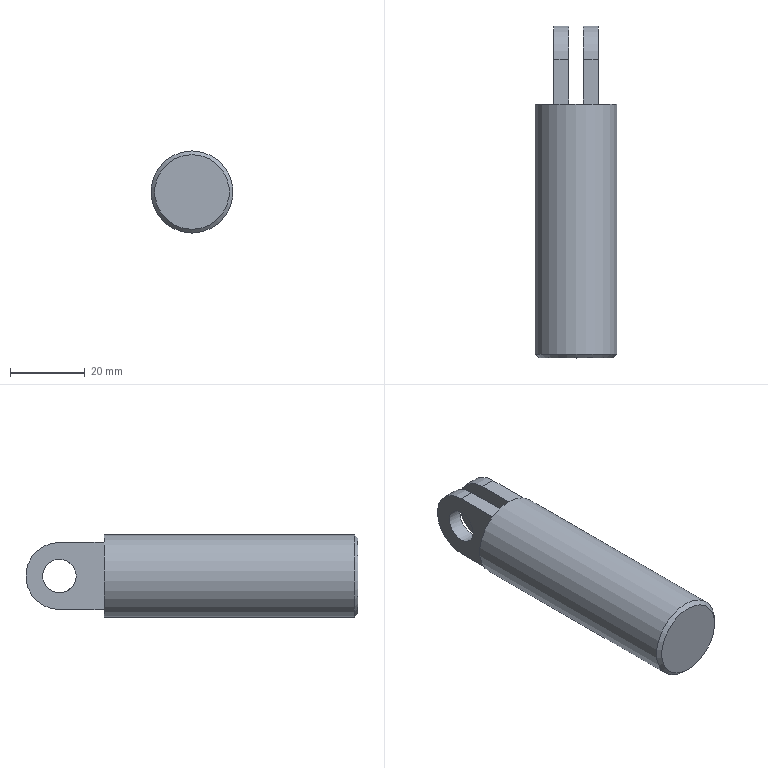Component | NX | PLUNGER | 1 solid | 16 faces | box 22 x 89 x 22 mm | volume 28052 mm3 | plane 10 | cylinder 5 | cone 1 | commonest cylinder face diameters 18 x2 9 x2 22 x1
STEP:
#1=CARTESIAN_POINT('',(0.,0.,0.));
#2=DIRECTION('',(0.,0.,1.));
#3=DIRECTION('',(1.,0.,0.));
#4=AXIS2_PLACEMENT_3D('',#1,#2,#3);
#5=CARTESIAN_POINT('',(-2.,64.5,19.75));
#6=VERTEX_POINT('',#5);
#7=CARTESIAN_POINT('',(-2.,52.5,19.75));
#8=VERTEX_POINT('',#7);
#9=CARTESIAN_POINT('',(-2.,64.5,19.75));
#10=DIRECTION('',(0.,-1.,-0.));
#11=VECTOR('',#10,1.);
#12=LINE('',#9,#11);
#13=CARTESIAN_POINT('',(-6.,64.5,19.75));
#14=DIRECTION('',(0.,-0.,1.));
#15=DIRECTION('',(0.,-1.,-0.));
#16=AXIS2_PLACEMENT_3D('',#13,#14,#15);
#17=PLANE('',#16);
#18=CARTESIAN_POINT('',(0.,4.));
#19=DIRECTION('',(1.,0.));
#20=VECTOR('',#19,1.);
#21=LINE('',#18,#20);
#22=(GEOMETRIC_REPRESENTATION_CONTEXT(2)PARAMETRIC_REPRESENTATION_CONTEXT()REPRESENTATION_CONTEXT('',''));
#23=DEFINITIONAL_REPRESENTATION('',(#21),#22);
#24=PCURVE('',#17,#23);
#25=CARTESIAN_POINT('',(-2.,76.,27.55));
#26=DIRECTION('',(-1.,0.,0.));
#27=DIRECTION('',(0.,-1.,0.));
#28=AXIS2_PLACEMENT_3D('',#25,#26,#27);
#29=PLANE('',#28);
#30=CARTESIAN_POINT('',(11.5,-7.8));
#31=DIRECTION('',(1.,-0.));
#32=VECTOR('',#31,1.);
#33=LINE('',#30,#32);
#34=(GEOMETRIC_REPRESENTATION_CONTEXT(2)PARAMETRIC_REPRESENTATION_CONTEXT()REPRESENTATION_CONTEXT('',''));
#35=DEFINITIONAL_REPRESENTATION('',(#33),#34);
#36=PCURVE('',#29,#35);
#37=SURFACE_CURVE('',#12,(#24,#36),.PCURVE_S1.);
#38=EDGE_CURVE('',#6,#8,#37,.T.);
#39=ORIENTED_EDGE('',*,*,#38,.F.);
#40=CARTESIAN_POINT('',(-6.,64.5,19.75));
#41=VERTEX_POINT('',#40);
#42=CARTESIAN_POINT('',(-6.,64.5,19.75));
#43=DIRECTION('',(1.,0.,0.));
#44=VECTOR('',#43,1.);
#45=LINE('',#42,#44);
#46=CARTESIAN_POINT('',(0.,0.));
#47=DIRECTION('',(0.,1.));
#48=VECTOR('',#47,1.);
#49=LINE('',#46,#48);
#50=(GEOMETRIC_REPRESENTATION_CONTEXT(2)PARAMETRIC_REPRESENTATION_CONTEXT()REPRESENTATION_CONTEXT('',''));
#51=DEFINITIONAL_REPRESENTATION('',(#49),#50);
#52=PCURVE('',#17,#51);
#53=CARTESIAN_POINT('',(-6.,64.5,10.75));
#54=DIRECTION('',(1.,0.,0.));
#55=DIRECTION('',(0.,1.,0.));
#56=AXIS2_PLACEMENT_3D('',#53,#54,#55);
#57=CYLINDRICAL_SURFACE('',#56,9.);
#58=CARTESIAN_POINT('',(7.854,0.));
#59=DIRECTION('',(0.,1.));
#60=VECTOR('',#59,1.);
#61=LINE('',#58,#60);
#62=(GEOMETRIC_REPRESENTATION_CONTEXT(2)PARAMETRIC_REPRESENTATION_CONTEXT()REPRESENTATION_CONTEXT('',''));
#63=DEFINITIONAL_REPRESENTATION('',(#61),#62);
#64=PCURVE('',#57,#63);
#65=SURFACE_CURVE('',#45,(#52,#64),.PCURVE_S1.);
#66=EDGE_CURVE('',#41,#6,#65,.T.);
#67=ORIENTED_EDGE('',*,*,#66,.F.);
#68=CARTESIAN_POINT('',(-6.,52.5,19.75));
#69=VERTEX_POINT('',#68);
#70=CARTESIAN_POINT('',(-6.,64.5,19.75));
#71=DIRECTION('',(0.,-1.,-0.));
#72=VECTOR('',#71,1.);
#73=LINE('',#70,#72);
#74=CARTESIAN_POINT('',(0.,0.));
#75=DIRECTION('',(1.,0.));
#76=VECTOR('',#75,1.);
#77=LINE('',#74,#76);
#78=(GEOMETRIC_REPRESENTATION_CONTEXT(2)PARAMETRIC_REPRESENTATION_CONTEXT()REPRESENTATION_CONTEXT('',''));
#79=DEFINITIONAL_REPRESENTATION('',(#77),#78);
#80=PCURVE('',#17,#79);
#81=CARTESIAN_POINT('',(-6.,64.5,10.75));
#82=DIRECTION('',(1.,0.,0.));
#83=DIRECTION('',(0.,1.,0.));
#84=AXIS2_PLACEMENT_3D('',#81,#82,#83);
#85=PLANE('',#84);
#86=CARTESIAN_POINT('',(0.,9.));
#87=DIRECTION('',(-1.,-0.));
#88=VECTOR('',#87,1.);
#89=LINE('',#86,#88);
#90=(GEOMETRIC_REPRESENTATION_CONTEXT(2)PARAMETRIC_REPRESENTATION_CONTEXT()REPRESENTATION_CONTEXT('',''));
#91=DEFINITIONAL_REPRESENTATION('',(#89),#90);
#92=PCURVE('',#85,#91);
#93=SURFACE_CURVE('',#73,(#80,#92),.PCURVE_S1.);
#94=EDGE_CURVE('',#41,#69,#93,.T.);
#95=ORIENTED_EDGE('',*,*,#94,.T.);
#96=CARTESIAN_POINT('',(-6.,52.5,19.75));
#97=DIRECTION('',(1.,0.,0.));
#98=VECTOR('',#97,1.);
#99=LINE('',#96,#98);
#100=CARTESIAN_POINT('',(12.,0.));
#101=DIRECTION('',(0.,1.));
#102=VECTOR('',#101,1.);
#103=LINE('',#100,#102);
#104=(GEOMETRIC_REPRESENTATION_CONTEXT(2)PARAMETRIC_REPRESENTATION_CONTEXT()REPRESENTATION_CONTEXT('',''));
#105=DEFINITIONAL_REPRESENTATION('',(#103),#104);
#106=PCURVE('',#17,#105);
#107=CARTESIAN_POINT('',(-0.,52.5,10.75));
#108=DIRECTION('',(0.,1.,0.));
#109=DIRECTION('',(0.,0.,1.));
#110=AXIS2_PLACEMENT_3D('',#107,#108,#109);
#111=PLANE('',#110);
#112=CARTESIAN_POINT('',(9.,-6.));
#113=DIRECTION('',(0.,1.));
#114=VECTOR('',#113,1.);
#115=LINE('',#112,#114);
#116=(GEOMETRIC_REPRESENTATION_CONTEXT(2)PARAMETRIC_REPRESENTATION_CONTEXT()REPRESENTATION_CONTEXT('',''));
#117=DEFINITIONAL_REPRESENTATION('',(#115),#116);
#118=PCURVE('',#111,#117);
#119=SURFACE_CURVE('',#99,(#106,#118),.PCURVE_S1.);
#120=EDGE_CURVE('',#69,#8,#119,.T.);
#121=ORIENTED_EDGE('',*,*,#120,.T.);
#122=EDGE_LOOP('',(#39,#67,#95,#121));
#123=FACE_BOUND('',#122,.T.);
#124=ADVANCED_FACE('',(#123),#17,.T.);
#125=CARTESIAN_POINT('',(-2.,52.5,1.75));
#126=VERTEX_POINT('',#125);
#127=CARTESIAN_POINT('',(-2.,64.5,1.75));
#128=VERTEX_POINT('',#127);
#129=CARTESIAN_POINT('',(-2.,52.5,1.75));
#130=DIRECTION('',(0.,1.,-0.));
#131=VECTOR('',#130,1.);
#132=LINE('',#129,#131);
#133=CARTESIAN_POINT('',(-6.,52.5,1.75));
#134=DIRECTION('',(0.,-0.,-1.));
#135=DIRECTION('',(0.,1.,-0.));
#136=AXIS2_PLACEMENT_3D('',#133,#134,#135);
#137=PLANE('',#136);
#138=CARTESIAN_POINT('',(0.,4.));
#139=DIRECTION('',(1.,0.));
#140=VECTOR('',#139,1.);
#141=LINE('',#138,#140);
#142=(GEOMETRIC_REPRESENTATION_CONTEXT(2)PARAMETRIC_REPRESENTATION_CONTEXT()REPRESENTATION_CONTEXT('',''));
#143=DEFINITIONAL_REPRESENTATION('',(#141),#142);
#144=PCURVE('',#137,#143);
#145=CARTESIAN_POINT('',(23.5,-25.8));
#146=DIRECTION('',(-1.,-0.));
#147=VECTOR('',#146,1.);
#148=LINE('',#145,#147);
#149=(GEOMETRIC_REPRESENTATION_CONTEXT(2)PARAMETRIC_REPRESENTATION_CONTEXT()REPRESENTATION_CONTEXT('',''));
#150=DEFINITIONAL_REPRESENTATION('',(#148),#149);
#151=PCURVE('',#29,#150);
#152=SURFACE_CURVE('',#132,(#144,#151),.PCURVE_S1.);
#153=EDGE_CURVE('',#126,#128,#152,.T.);
#154=ORIENTED_EDGE('',*,*,#153,.F.);
#155=CARTESIAN_POINT('',(-6.,52.5,1.75));
#156=VERTEX_POINT('',#155);
#157=CARTESIAN_POINT('',(-6.,52.5,1.75));
#158=DIRECTION('',(1.,0.,0.));
#159=VECTOR('',#158,1.);
#160=LINE('',#157,#159);
#161=CARTESIAN_POINT('',(0.,0.));
#162=DIRECTION('',(0.,1.));
#163=VECTOR('',#162,1.);
#164=LINE('',#161,#163);
#165=(GEOMETRIC_REPRESENTATION_CONTEXT(2)PARAMETRIC_REPRESENTATION_CONTEXT()REPRESENTATION_CONTEXT('',''));
#166=DEFINITIONAL_REPRESENTATION('',(#164),#165);
#167=PCURVE('',#137,#166);
#168=CARTESIAN_POINT('',(-9.,-6.));
#169=DIRECTION('',(0.,1.));
#170=VECTOR('',#169,1.);
#171=LINE('',#168,#170);
#172=(GEOMETRIC_REPRESENTATION_CONTEXT(2)PARAMETRIC_REPRESENTATION_CONTEXT()REPRESENTATION_CONTEXT('',''));
#173=DEFINITIONAL_REPRESENTATION('',(#171),#172);
#174=PCURVE('',#111,#173);
#175=SURFACE_CURVE('',#160,(#167,#174),.PCURVE_S1.);
#176=EDGE_CURVE('',#156,#126,#175,.T.);
#177=ORIENTED_EDGE('',*,*,#176,.F.);
#178=CARTESIAN_POINT('',(-6.,64.5,1.75));
#179=VERTEX_POINT('',#178);
#180=CARTESIAN_POINT('',(-6.,52.5,1.75));
#181=DIRECTION('',(0.,1.,-0.));
#182=VECTOR('',#181,1.);
#183=LINE('',#180,#182);
#184=CARTESIAN_POINT('',(0.,0.));
#185=DIRECTION('',(1.,0.));
#186=VECTOR('',#185,1.);
#187=LINE('',#184,#186);
#188=(GEOMETRIC_REPRESENTATION_CONTEXT(2)PARAMETRIC_REPRESENTATION_CONTEXT()REPRESENTATION_CONTEXT('',''));
#189=DEFINITIONAL_REPRESENTATION('',(#187),#188);
#190=PCURVE('',#137,#189);
#191=CARTESIAN_POINT('',(-12.,-9.));
#192=DIRECTION('',(1.,-0.));
#193=VECTOR('',#192,1.);
#194=LINE('',#191,#193);
#195=(GEOMETRIC_REPRESENTATION_CONTEXT(2)PARAMETRIC_REPRESENTATION_CONTEXT()REPRESENTATION_CONTEXT('',''));
#196=DEFINITIONAL_REPRESENTATION('',(#194),#195);
#197=PCURVE('',#85,#196);
#198=SURFACE_CURVE('',#183,(#190,#197),.PCURVE_S1.);
#199=EDGE_CURVE('',#156,#179,#198,.T.);
#200=ORIENTED_EDGE('',*,*,#199,.T.);
#201=CARTESIAN_POINT('',(-6.,64.5,1.75));
#202=DIRECTION('',(1.,0.,0.));
#203=VECTOR('',#202,1.);
#204=LINE('',#201,#203);
#205=CARTESIAN_POINT('',(12.,0.));
#206=DIRECTION('',(0.,1.));
#207=VECTOR('',#206,1.);
#208=LINE('',#205,#207);
#209=(GEOMETRIC_REPRESENTATION_CONTEXT(2)PARAMETRIC_REPRESENTATION_CONTEXT()REPRESENTATION_CONTEXT('',''));
#210=DEFINITIONAL_REPRESENTATION('',(#208),#209);
#211=PCURVE('',#137,#210);
#212=CARTESIAN_POINT('',(4.712,0.));
#213=DIRECTION('',(0.,1.));
#214=VECTOR('',#213,1.);
#215=LINE('',#212,#214);
#216=(GEOMETRIC_REPRESENTATION_CONTEXT(2)PARAMETRIC_REPRESENTATION_CONTEXT()REPRESENTATION_CONTEXT('',''));
#217=DEFINITIONAL_REPRESENTATION('',(#215),#216);
#218=PCURVE('',#57,#217);
#219=SURFACE_CURVE('',#204,(#211,#218),.PCURVE_S1.);
#220=EDGE_CURVE('',#179,#128,#219,.T.);
#221=ORIENTED_EDGE('',*,*,#220,.T.);
#222=EDGE_LOOP('',(#154,#177,#200,#221));
#223=FACE_BOUND('',#222,.T.);
#224=ADVANCED_FACE('',(#223),#137,.T.);
#225=CARTESIAN_POINT('',(-2.,64.5,10.75));
#226=DIRECTION('',(1.,0.,0.));
#227=DIRECTION('',(0.,-1.,0.));
#228=AXIS2_PLACEMENT_3D('',#225,#226,#227);
#229=CIRCLE('',#228,9.);
#230=CARTESIAN_POINT('',(3.142,4.));
#231=DIRECTION('',(1.,0.));
#232=VECTOR('',#231,1.);
#233=LINE('',#230,#232);
#234=(GEOMETRIC_REPRESENTATION_CONTEXT(2)PARAMETRIC_REPRESENTATION_CONTEXT()REPRESENTATION_CONTEXT('',''));
#235=DEFINITIONAL_REPRESENTATION('',(#233),#234);
#236=PCURVE('',#57,#235);
#237=CARTESIAN_POINT('',(20.5,-16.8));
#238=CARTESIAN_POINT('',(20.5,-32.388));
#239=CARTESIAN_POINT('',(7.,-24.594));
#240=CARTESIAN_POINT('',(-6.5,-16.8));
#241=CARTESIAN_POINT('',(7.,-9.006));
#242=CARTESIAN_POINT('',(20.5,-1.212));
#243=CARTESIAN_POINT('',(20.5,-16.8));
#244=(BOUNDED_CURVE()B_SPLINE_CURVE(2,(#237,#238,#239,#240,#241,#242,#243),.UNSPECIFIED.,.T.,.F.)B_SPLINE_CURVE_WITH_KNOTS((1,2,2,2,2,1),(-2.094,0.,2.094,4.189,6.283,8.378),.UNSPECIFIED.)CURVE()GEOMETRIC_REPRESENTATION_ITEM()RATIONAL_B_SPLINE_CURVE((1.,0.5,1.,0.5,1.,0.5,1.))REPRESENTATION_ITEM(''));
#245=(GEOMETRIC_REPRESENTATION_CONTEXT(2)PARAMETRIC_REPRESENTATION_CONTEXT()REPRESENTATION_CONTEXT('',''));
#246=DEFINITIONAL_REPRESENTATION('',(#244),#245);
#247=PCURVE('',#29,#246);
#248=SURFACE_CURVE('',#229,(#236,#247),.PCURVE_S1.);
#249=EDGE_CURVE('',#128,#6,#248,.T.);
#250=ORIENTED_EDGE('',*,*,#249,.F.);
#251=ORIENTED_EDGE('',*,*,#220,.F.);
#252=CARTESIAN_POINT('',(-6.,64.5,10.75));
#253=DIRECTION('',(1.,0.,0.));
#254=DIRECTION('',(0.,0.,1.));
#255=AXIS2_PLACEMENT_3D('',#252,#253,#254);
#256=CIRCLE('',#255,9.);
#257=CARTESIAN_POINT('',(1.571,0.));
#258=DIRECTION('',(1.,0.));
#259=VECTOR('',#258,1.);
#260=LINE('',#257,#259);
#261=(GEOMETRIC_REPRESENTATION_CONTEXT(2)PARAMETRIC_REPRESENTATION_CONTEXT()REPRESENTATION_CONTEXT('',''));
#262=DEFINITIONAL_REPRESENTATION('',(#260),#261);
#263=PCURVE('',#57,#262);
#264=CARTESIAN_POINT('',(0.,0.));
#265=DIRECTION('',(0.,1.));
#266=AXIS2_PLACEMENT_2D('',#264,#265);
#267=CIRCLE('',#266,9.);
#268=(GEOMETRIC_REPRESENTATION_CONTEXT(2)PARAMETRIC_REPRESENTATION_CONTEXT()REPRESENTATION_CONTEXT('',''));
#269=DEFINITIONAL_REPRESENTATION('',(#267),#268);
#270=PCURVE('',#85,#269);
#271=SURFACE_CURVE('',#256,(#263,#270),.PCURVE_S1.);
#272=EDGE_CURVE('',#179,#41,#271,.T.);
#273=ORIENTED_EDGE('',*,*,#272,.T.);
#274=ORIENTED_EDGE('',*,*,#66,.T.);
#275=EDGE_LOOP('',(#250,#251,#273,#274));
#276=FACE_BOUND('',#275,.T.);
#277=ADVANCED_FACE('',(#276),#57,.T.);
#278=CARTESIAN_POINT('',(2.,52.5,19.75));
#279=VERTEX_POINT('',#278);
#280=CARTESIAN_POINT('',(6.,52.5,19.75));
#281=VERTEX_POINT('',#280);
#282=CARTESIAN_POINT('',(-6.,52.5,19.75));
#283=DIRECTION('',(1.,0.,0.));
#284=VECTOR('',#283,1.);
#285=LINE('',#282,#284);
#286=CARTESIAN_POINT('',(9.,-6.));
#287=DIRECTION('',(0.,1.));
#288=VECTOR('',#287,1.);
#289=LINE('',#286,#288);
#290=(GEOMETRIC_REPRESENTATION_CONTEXT(2)PARAMETRIC_REPRESENTATION_CONTEXT()REPRESENTATION_CONTEXT('',''));
#291=DEFINITIONAL_REPRESENTATION('',(#289),#290);
#292=PCURVE('',#111,#291);
#293=CARTESIAN_POINT('',(-6.,64.5,19.75));
#294=DIRECTION('',(0.,-0.,1.));
#295=DIRECTION('',(0.,-1.,-0.));
#296=AXIS2_PLACEMENT_3D('',#293,#294,#295);
#297=PLANE('',#296);
#298=CARTESIAN_POINT('',(12.,0.));
#299=DIRECTION('',(0.,1.));
#300=VECTOR('',#299,1.);
#301=LINE('',#298,#300);
#302=(GEOMETRIC_REPRESENTATION_CONTEXT(2)PARAMETRIC_REPRESENTATION_CONTEXT()REPRESENTATION_CONTEXT('',''));
#303=DEFINITIONAL_REPRESENTATION('',(#301),#302);
#304=PCURVE('',#297,#303);
#305=SURFACE_CURVE('',#285,(#292,#304),.PCURVE_S1.);
#306=EDGE_CURVE('',#279,#281,#305,.T.);
#307=ORIENTED_EDGE('',*,*,#306,.F.);
#308=CARTESIAN_POINT('',(2.,52.5,1.75));
#309=VERTEX_POINT('',#308);
#310=CARTESIAN_POINT('',(2.,52.5,-6.05));
#311=DIRECTION('',(0.,0.,1.));
#312=VECTOR('',#311,1.);
#313=LINE('',#310,#312);
#314=CARTESIAN_POINT('',(-16.8,2.));
#315=DIRECTION('',(1.,0.));
#316=VECTOR('',#315,1.);
#317=LINE('',#314,#316);
#318=(GEOMETRIC_REPRESENTATION_CONTEXT(2)PARAMETRIC_REPRESENTATION_CONTEXT()REPRESENTATION_CONTEXT('',''));
#319=DEFINITIONAL_REPRESENTATION('',(#317),#318);
#320=PCURVE('',#111,#319);
#321=CARTESIAN_POINT('',(2.,76.,-6.05));
#322=DIRECTION('',(1.,0.,0.));
#323=DIRECTION('',(0.,1.,0.));
#324=AXIS2_PLACEMENT_3D('',#321,#322,#323);
#325=PLANE('',#324);
#326=CARTESIAN_POINT('',(-23.5,0.));
#327=DIRECTION('',(0.,1.));
#328=VECTOR('',#327,1.);
#329=LINE('',#326,#328);
#330=(GEOMETRIC_REPRESENTATION_CONTEXT(2)PARAMETRIC_REPRESENTATION_CONTEXT()REPRESENTATION_CONTEXT('',''));
#331=DEFINITIONAL_REPRESENTATION('',(#329),#330);
#332=PCURVE('',#325,#331);
#333=SURFACE_CURVE('',#313,(#320,#332),.PCURVE_S1.);
#334=EDGE_CURVE('',#309,#279,#333,.T.);
#335=ORIENTED_EDGE('',*,*,#334,.F.);
#336=CARTESIAN_POINT('',(6.,52.5,1.75));
#337=VERTEX_POINT('',#336);
#338=CARTESIAN_POINT('',(-6.,52.5,1.75));
#339=DIRECTION('',(1.,0.,0.));
#340=VECTOR('',#339,1.);
#341=LINE('',#338,#340);
#342=CARTESIAN_POINT('',(-9.,-6.));
#343=DIRECTION('',(0.,1.));
#344=VECTOR('',#343,1.);
#345=LINE('',#342,#344);
#346=(GEOMETRIC_REPRESENTATION_CONTEXT(2)PARAMETRIC_REPRESENTATION_CONTEXT()REPRESENTATION_CONTEXT('',''));
#347=DEFINITIONAL_REPRESENTATION('',(#345),#346);
#348=PCURVE('',#111,#347);
#349=CARTESIAN_POINT('',(-6.,52.5,1.75));
#350=DIRECTION('',(0.,-0.,-1.));
#351=DIRECTION('',(0.,1.,-0.));
#352=AXIS2_PLACEMENT_3D('',#349,#350,#351);
#353=PLANE('',#352);
#354=CARTESIAN_POINT('',(0.,0.));
#355=DIRECTION('',(0.,1.));
#356=VECTOR('',#355,1.);
#357=LINE('',#354,#356);
#358=(GEOMETRIC_REPRESENTATION_CONTEXT(2)PARAMETRIC_REPRESENTATION_CONTEXT()REPRESENTATION_CONTEXT('',''));
#359=DEFINITIONAL_REPRESENTATION('',(#357),#358);
#360=PCURVE('',#353,#359);
#361=SURFACE_CURVE('',#341,(#348,#360),.PCURVE_S1.);
#362=EDGE_CURVE('',#309,#337,#361,.T.);
#363=ORIENTED_EDGE('',*,*,#362,.T.);
#364=CARTESIAN_POINT('',(6.,52.5,10.75));
#365=DIRECTION('',(0.,0.,-1.));
#366=VECTOR('',#365,1.);
#367=LINE('',#364,#366);
#368=CARTESIAN_POINT('',(0.,6.));
#369=DIRECTION('',(-1.,0.));
#370=VECTOR('',#369,1.);
#371=LINE('',#368,#370);
#372=(GEOMETRIC_REPRESENTATION_CONTEXT(2)PARAMETRIC_REPRESENTATION_CONTEXT()REPRESENTATION_CONTEXT('',''));
#373=DEFINITIONAL_REPRESENTATION('',(#371),#372);
#374=PCURVE('',#111,#373);
#375=CARTESIAN_POINT('',(6.,64.5,10.75));
#376=DIRECTION('',(1.,0.,0.));
#377=DIRECTION('',(0.,1.,0.));
#378=AXIS2_PLACEMENT_3D('',#375,#376,#377);
#379=PLANE('',#378);
#380=CARTESIAN_POINT('',(-12.,0.));
#381=DIRECTION('',(0.,-1.));
#382=VECTOR('',#381,1.);
#383=LINE('',#380,#382);
#384=(GEOMETRIC_REPRESENTATION_CONTEXT(2)PARAMETRIC_REPRESENTATION_CONTEXT()REPRESENTATION_CONTEXT('',''));
#385=DEFINITIONAL_REPRESENTATION('',(#383),#384);
#386=PCURVE('',#379,#385);
#387=SURFACE_CURVE('',#367,(#374,#386),.PCURVE_S1.);
#388=EDGE_CURVE('',#281,#337,#387,.T.);
#389=ORIENTED_EDGE('',*,*,#388,.F.);
#390=EDGE_LOOP('',(#307,#335,#363,#389));
#391=FACE_BOUND('',#390,.T.);
#392=CARTESIAN_POINT('',(-2.,52.5,27.55));
#393=DIRECTION('',(0.,0.,-1.));
#394=VECTOR('',#393,1.);
#395=LINE('',#392,#394);
#396=CARTESIAN_POINT('',(16.8,-2.));
#397=DIRECTION('',(-1.,0.));
#398=VECTOR('',#397,1.);
#399=LINE('',#396,#398);
#400=(GEOMETRIC_REPRESENTATION_CONTEXT(2)PARAMETRIC_REPRESENTATION_CONTEXT()REPRESENTATION_CONTEXT('',''));
#401=DEFINITIONAL_REPRESENTATION('',(#399),#400);
#402=PCURVE('',#111,#401);
#403=CARTESIAN_POINT('',(23.5,0.));
#404=DIRECTION('',(0.,-1.));
#405=VECTOR('',#404,1.);
#406=LINE('',#403,#405);
#407=(GEOMETRIC_REPRESENTATION_CONTEXT(2)PARAMETRIC_REPRESENTATION_CONTEXT()REPRESENTATION_CONTEXT('',''));
#408=DEFINITIONAL_REPRESENTATION('',(#406),#407);
#409=PCURVE('',#29,#408);
#410=SURFACE_CURVE('',#395,(#402,#409),.PCURVE_S1.);
#411=EDGE_CURVE('',#8,#126,#410,.T.);
#412=ORIENTED_EDGE('',*,*,#411,.F.);
#413=ORIENTED_EDGE('',*,*,#120,.F.);
#414=CARTESIAN_POINT('',(-6.,52.5,19.75));
#415=DIRECTION('',(0.,0.,-1.));
#416=VECTOR('',#415,1.);
#417=LINE('',#414,#416);
#418=CARTESIAN_POINT('',(9.,-6.));
#419=DIRECTION('',(-1.,0.));
#420=VECTOR('',#419,1.);
#421=LINE('',#418,#420);
#422=(GEOMETRIC_REPRESENTATION_CONTEXT(2)PARAMETRIC_REPRESENTATION_CONTEXT()REPRESENTATION_CONTEXT('',''));
#423=DEFINITIONAL_REPRESENTATION('',(#421),#422);
#424=PCURVE('',#111,#423);
#425=CARTESIAN_POINT('',(-12.,9.));
#426=DIRECTION('',(0.,-1.));
#427=VECTOR('',#426,1.);
#428=LINE('',#425,#427);
#429=(GEOMETRIC_REPRESENTATION_CONTEXT(2)PARAMETRIC_REPRESENTATION_CONTEXT()REPRESENTATION_CONTEXT('',''));
#430=DEFINITIONAL_REPRESENTATION('',(#428),#429);
#431=PCURVE('',#85,#430);
#432=SURFACE_CURVE('',#417,(#424,#431),.PCURVE_S1.);
#433=EDGE_CURVE('',#69,#156,#432,.T.);
#434=ORIENTED_EDGE('',*,*,#433,.T.);
#435=ORIENTED_EDGE('',*,*,#176,.T.);
#436=EDGE_LOOP('',(#412,#413,#434,#435));
#437=FACE_BOUND('',#436,.T.);
#438=CARTESIAN_POINT('',(-0.,52.5,21.75));
#439=VERTEX_POINT('',#438);
#440=CARTESIAN_POINT('',(-0.,52.5,10.75));
#441=DIRECTION('',(0.,-1.,0.));
#442=DIRECTION('',(0.,0.,1.));
#443=AXIS2_PLACEMENT_3D('',#440,#441,#442);
#444=CIRCLE('',#443,11.);
#445=CARTESIAN_POINT('',(11.,0.));
#446=CARTESIAN_POINT('',(11.,-19.053));
#447=CARTESIAN_POINT('',(-5.5,-9.526));
#448=CARTESIAN_POINT('',(-22.,-0.));
#449=CARTESIAN_POINT('',(-5.5,9.526));
#450=CARTESIAN_POINT('',(11.,19.053));
#451=CARTESIAN_POINT('',(11.,0.));
#452=(BOUNDED_CURVE()B_SPLINE_CURVE(2,(#445,#446,#447,#448,#449,#450,#451),.UNSPECIFIED.,.T.,.F.)B_SPLINE_CURVE_WITH_KNOTS((1,2,2,2,2,1),(-2.094,0.,2.094,4.189,6.283,8.378),.UNSPECIFIED.)CURVE()GEOMETRIC_REPRESENTATION_ITEM()RATIONAL_B_SPLINE_CURVE((1.,0.5,1.,0.5,1.,0.5,1.))REPRESENTATION_ITEM(''));
#453=(GEOMETRIC_REPRESENTATION_CONTEXT(2)PARAMETRIC_REPRESENTATION_CONTEXT()REPRESENTATION_CONTEXT('',''));
#454=DEFINITIONAL_REPRESENTATION('',(#452),#453);
#455=PCURVE('',#111,#454);
#456=CARTESIAN_POINT('',(-0.,-15.5,10.75));
#457=DIRECTION('',(0.,1.,0.));
#458=DIRECTION('',(0.,0.,1.));
#459=AXIS2_PLACEMENT_3D('',#456,#457,#458);
#460=CYLINDRICAL_SURFACE('',#459,11.);
#461=CARTESIAN_POINT('',(6.283,68.));
#462=DIRECTION('',(-1.,0.));
#463=VECTOR('',#462,1.);
#464=LINE('',#461,#463);
#465=(GEOMETRIC_REPRESENTATION_CONTEXT(2)PARAMETRIC_REPRESENTATION_CONTEXT()REPRESENTATION_CONTEXT('',''));
#466=DEFINITIONAL_REPRESENTATION('',(#464),#465);
#467=PCURVE('',#460,#466);
#468=SURFACE_CURVE('',#444,(#455,#467),.PCURVE_S1.);
#469=EDGE_CURVE('',#439,#439,#468,.T.);
#470=ORIENTED_EDGE('',*,*,#469,.F.);
#471=EDGE_LOOP('',(#470));
#472=FACE_BOUND('',#471,.T.);
#473=ADVANCED_FACE('',(#391,#437,#472),#111,.T.);
#474=CARTESIAN_POINT('',(-0.,-15.5,0.75));
#475=VERTEX_POINT('',#474);
#476=CARTESIAN_POINT('',(-0.,-15.5,10.75));
#477=DIRECTION('',(0.,-1.,0.));
#478=DIRECTION('',(0.,0.,-1.));
#479=AXIS2_PLACEMENT_3D('',#476,#477,#478);
#480=CIRCLE('',#479,10.);
#481=CARTESIAN_POINT('',(-0.,-15.5,10.75));
#482=DIRECTION('',(0.,-1.,0.));
#483=DIRECTION('',(0.,0.,-1.));
#484=AXIS2_PLACEMENT_3D('',#481,#482,#483);
#485=PLANE('',#484);
#486=CARTESIAN_POINT('',(0.,0.));
#487=DIRECTION('',(1.,0.));
#488=AXIS2_PLACEMENT_2D('',#486,#487);
#489=CIRCLE('',#488,10.);
#490=(GEOMETRIC_REPRESENTATION_CONTEXT(2)PARAMETRIC_REPRESENTATION_CONTEXT()REPRESENTATION_CONTEXT('',''));
#491=DEFINITIONAL_REPRESENTATION('',(#489),#490);
#492=PCURVE('',#485,#491);
#493=CARTESIAN_POINT('',(-0.,-14.5,10.75));
#494=DIRECTION('',(0.,1.,0.));
#495=DIRECTION('',(0.,0.,1.));
#496=AXIS2_PLACEMENT_3D('',#493,#494,#495);
#497=CONICAL_SURFACE('',#496,11.,0.7854);
#498=CARTESIAN_POINT('',(9.425,-1.));
#499=DIRECTION('',(-1.,0.));
#500=VECTOR('',#499,1.);
#501=LINE('',#498,#500);
#502=(GEOMETRIC_REPRESENTATION_CONTEXT(2)PARAMETRIC_REPRESENTATION_CONTEXT()REPRESENTATION_CONTEXT('',''));
#503=DEFINITIONAL_REPRESENTATION('',(#501),#502);
#504=PCURVE('',#497,#503);
#505=SURFACE_CURVE('',#480,(#492,#504),.PCURVE_S1.);
#506=EDGE_CURVE('',#475,#475,#505,.T.);
#507=ORIENTED_EDGE('',*,*,#506,.T.);
#508=EDGE_LOOP('',(#507));
#509=FACE_BOUND('',#508,.T.);
#510=ADVANCED_FACE('',(#509),#485,.T.);
#511=CARTESIAN_POINT('',(-0.,-14.5,-0.25));
#512=VERTEX_POINT('',#511);
#513=CARTESIAN_POINT('',(-0.,-14.5,21.75));
#514=VERTEX_POINT('',#513);
#515=CARTESIAN_POINT('',(-0.,-14.5,10.75));
#516=DIRECTION('',(0.,1.,0.));
#517=DIRECTION('',(0.,0.,-1.));
#518=AXIS2_PLACEMENT_3D('',#515,#516,#517);
#519=CIRCLE('',#518,11.);
#520=CARTESIAN_POINT('',(3.142,1.));
#521=DIRECTION('',(1.,0.));
#522=VECTOR('',#521,1.);
#523=LINE('',#520,#522);
#524=(GEOMETRIC_REPRESENTATION_CONTEXT(2)PARAMETRIC_REPRESENTATION_CONTEXT()REPRESENTATION_CONTEXT('',''));
#525=DEFINITIONAL_REPRESENTATION('',(#523),#524);
#526=PCURVE('',#460,#525);
#527=CARTESIAN_POINT('',(3.142,0.));
#528=DIRECTION('',(1.,0.));
#529=VECTOR('',#528,1.);
#530=LINE('',#527,#529);
#531=(GEOMETRIC_REPRESENTATION_CONTEXT(2)PARAMETRIC_REPRESENTATION_CONTEXT()REPRESENTATION_CONTEXT('',''));
#532=DEFINITIONAL_REPRESENTATION('',(#530),#531);
#533=PCURVE('',#497,#532);
#534=SURFACE_CURVE('',#519,(#526,#533),.PCURVE_S1.);
#535=EDGE_CURVE('',#512,#514,#534,.T.);
#536=ORIENTED_EDGE('',*,*,#535,.T.);
#537=CARTESIAN_POINT('',(-0.,-14.5,21.75));
#538=CARTESIAN_POINT('',(-0.,52.5,21.75));
#539=B_SPLINE_CURVE_WITH_KNOTS('',1,(#537,#538),.UNSPECIFIED.,.F.,.F.,(2,2),(1.,68.),.PIECEWISE_BEZIER_KNOTS.);
#540=CARTESIAN_POINT('',(6.283,0.));
#541=DIRECTION('',(0.,1.));
#542=VECTOR('',#541,1.);
#543=LINE('',#540,#542);
#544=(GEOMETRIC_REPRESENTATION_CONTEXT(2)PARAMETRIC_REPRESENTATION_CONTEXT()REPRESENTATION_CONTEXT('',''));
#545=DEFINITIONAL_REPRESENTATION('',(#543),#544);
#546=PCURVE('',#460,#545);
#547=CARTESIAN_POINT('',(0.,0.));
#548=DIRECTION('',(0.,1.));
#549=VECTOR('',#548,1.);
#550=LINE('',#547,#549);
#551=(GEOMETRIC_REPRESENTATION_CONTEXT(2)PARAMETRIC_REPRESENTATION_CONTEXT()REPRESENTATION_CONTEXT('',''));
#552=DEFINITIONAL_REPRESENTATION('',(#550),#551);
#553=PCURVE('',#460,#552);
#554=SEAM_CURVE('',#539,(#546,#553),.PCURVE_S1.);
#555=EDGE_CURVE('',#514,#439,#554,.T.);
#556=ORIENTED_EDGE('',*,*,#555,.T.);
#557=ORIENTED_EDGE('',*,*,#469,.T.);
#558=ORIENTED_EDGE('',*,*,#555,.F.);
#559=CARTESIAN_POINT('',(-0.,-14.5,10.75));
#560=DIRECTION('',(0.,1.,0.));
#561=DIRECTION('',(0.,0.,-1.));
#562=AXIS2_PLACEMENT_3D('',#559,#560,#561);
#563=CIRCLE('',#562,11.);
#564=CARTESIAN_POINT('',(-3.142,1.));
#565=DIRECTION('',(1.,0.));
#566=VECTOR('',#565,1.);
#567=LINE('',#564,#566);
#568=(GEOMETRIC_REPRESENTATION_CONTEXT(2)PARAMETRIC_REPRESENTATION_CONTEXT()REPRESENTATION_CONTEXT('',''));
#569=DEFINITIONAL_REPRESENTATION('',(#567),#568);
#570=PCURVE('',#460,#569);
#571=CARTESIAN_POINT('',(3.142,0.));
#572=DIRECTION('',(1.,0.));
#573=VECTOR('',#572,1.);
#574=LINE('',#571,#573);
#575=(GEOMETRIC_REPRESENTATION_CONTEXT(2)PARAMETRIC_REPRESENTATION_CONTEXT()REPRESENTATION_CONTEXT('',''));
#576=DEFINITIONAL_REPRESENTATION('',(#574),#575);
#577=PCURVE('',#497,#576);
#578=SURFACE_CURVE('',#563,(#570,#577),.PCURVE_S1.);
#579=EDGE_CURVE('',#514,#512,#578,.T.);
#580=ORIENTED_EDGE('',*,*,#579,.T.);
#581=EDGE_LOOP('',(#536,#556,#557,#558,#580));
#582=FACE_BOUND('',#581,.T.);
#583=ADVANCED_FACE('',(#582),#460,.T.);
#584=CARTESIAN_POINT('',(2.,64.5,19.75));
#585=VERTEX_POINT('',#584);
#586=CARTESIAN_POINT('',(2.,64.5,19.75));
#587=DIRECTION('',(0.,1.,0.));
#588=VECTOR('',#587,1.);
#589=LINE('',#586,#588);
#590=CARTESIAN_POINT('',(0.,8.));
#591=DIRECTION('',(-1.,0.));
#592=VECTOR('',#591,1.);
#593=LINE('',#590,#592);
#594=(GEOMETRIC_REPRESENTATION_CONTEXT(2)PARAMETRIC_REPRESENTATION_CONTEXT()REPRESENTATION_CONTEXT('',''));
#595=DEFINITIONAL_REPRESENTATION('',(#593),#594);
#596=PCURVE('',#297,#595);
#597=CARTESIAN_POINT('',(-11.5,25.8));
#598=DIRECTION('',(1.,0.));
#599=VECTOR('',#598,1.);
#600=LINE('',#597,#599);
#601=(GEOMETRIC_REPRESENTATION_CONTEXT(2)PARAMETRIC_REPRESENTATION_CONTEXT()REPRESENTATION_CONTEXT('',''));
#602=DEFINITIONAL_REPRESENTATION('',(#600),#601);
#603=PCURVE('',#325,#602);
#604=SURFACE_CURVE('',#589,(#596,#603),.PCURVE_S1.);
#605=EDGE_CURVE('',#279,#585,#604,.T.);
#606=ORIENTED_EDGE('',*,*,#605,.F.);
#607=ORIENTED_EDGE('',*,*,#306,.T.);
#608=CARTESIAN_POINT('',(6.,64.5,19.75));
#609=VERTEX_POINT('',#608);
#610=CARTESIAN_POINT('',(6.,64.5,19.75));
#611=DIRECTION('',(0.,-1.,-0.));
#612=VECTOR('',#611,1.);
#613=LINE('',#610,#612);
#614=CARTESIAN_POINT('',(0.,12.));
#615=DIRECTION('',(1.,0.));
#616=VECTOR('',#615,1.);
#617=LINE('',#614,#616);
#618=(GEOMETRIC_REPRESENTATION_CONTEXT(2)PARAMETRIC_REPRESENTATION_CONTEXT()REPRESENTATION_CONTEXT('',''));
#619=DEFINITIONAL_REPRESENTATION('',(#617),#618);
#620=PCURVE('',#297,#619);
#621=CARTESIAN_POINT('',(0.,9.));
#622=DIRECTION('',(-1.,-0.));
#623=VECTOR('',#622,1.);
#624=LINE('',#621,#623);
#625=(GEOMETRIC_REPRESENTATION_CONTEXT(2)PARAMETRIC_REPRESENTATION_CONTEXT()REPRESENTATION_CONTEXT('',''));
#626=DEFINITIONAL_REPRESENTATION('',(#624),#625);
#627=PCURVE('',#379,#626);
#628=SURFACE_CURVE('',#613,(#620,#627),.PCURVE_S1.);
#629=EDGE_CURVE('',#609,#281,#628,.T.);
#630=ORIENTED_EDGE('',*,*,#629,.F.);
#631=CARTESIAN_POINT('',(-6.,64.5,19.75));
#632=DIRECTION('',(1.,0.,0.));
#633=VECTOR('',#632,1.);
#634=LINE('',#631,#633);
#635=CARTESIAN_POINT('',(0.,0.));
#636=DIRECTION('',(0.,1.));
#637=VECTOR('',#636,1.);
#638=LINE('',#635,#637);
#639=(GEOMETRIC_REPRESENTATION_CONTEXT(2)PARAMETRIC_REPRESENTATION_CONTEXT()REPRESENTATION_CONTEXT('',''));
#640=DEFINITIONAL_REPRESENTATION('',(#638),#639);
#641=PCURVE('',#297,#640);
#642=CARTESIAN_POINT('',(-6.,64.5,10.75));
#643=DIRECTION('',(1.,0.,0.));
#644=DIRECTION('',(0.,1.,0.));
#645=AXIS2_PLACEMENT_3D('',#642,#643,#644);
#646=CYLINDRICAL_SURFACE('',#645,9.);
#647=CARTESIAN_POINT('',(1.571,0.));
#648=DIRECTION('',(0.,1.));
#649=VECTOR('',#648,1.);
#650=LINE('',#647,#649);
#651=(GEOMETRIC_REPRESENTATION_CONTEXT(2)PARAMETRIC_REPRESENTATION_CONTEXT()REPRESENTATION_CONTEXT('',''));
#652=DEFINITIONAL_REPRESENTATION('',(#650),#651);
#653=PCURVE('',#646,#652);
#654=SURFACE_CURVE('',#634,(#641,#653),.PCURVE_S1.);
#655=EDGE_CURVE('',#585,#609,#654,.T.);
#656=ORIENTED_EDGE('',*,*,#655,.F.);
#657=EDGE_LOOP('',(#606,#607,#630,#656));
#658=FACE_BOUND('',#657,.T.);
#659=ADVANCED_FACE('',(#658),#297,.T.);
#660=CARTESIAN_POINT('',(2.,64.5,1.75));
#661=VERTEX_POINT('',#660);
#662=CARTESIAN_POINT('',(2.,52.5,1.75));
#663=DIRECTION('',(0.,-1.,0.));
#664=VECTOR('',#663,1.);
#665=LINE('',#662,#664);
#666=CARTESIAN_POINT('',(0.,8.));
#667=DIRECTION('',(-1.,0.));
#668=VECTOR('',#667,1.);
#669=LINE('',#666,#668);
#670=(GEOMETRIC_REPRESENTATION_CONTEXT(2)PARAMETRIC_REPRESENTATION_CONTEXT()REPRESENTATION_CONTEXT('',''));
#671=DEFINITIONAL_REPRESENTATION('',(#669),#670);
#672=PCURVE('',#353,#671);
#673=CARTESIAN_POINT('',(-23.5,7.8));
#674=DIRECTION('',(-1.,0.));
#675=VECTOR('',#674,1.);
#676=LINE('',#673,#675);
#677=(GEOMETRIC_REPRESENTATION_CONTEXT(2)PARAMETRIC_REPRESENTATION_CONTEXT()REPRESENTATION_CONTEXT('',''));
#678=DEFINITIONAL_REPRESENTATION('',(#676),#677);
#679=PCURVE('',#325,#678);
#680=SURFACE_CURVE('',#665,(#672,#679),.PCURVE_S1.);
#681=EDGE_CURVE('',#661,#309,#680,.T.);
#682=ORIENTED_EDGE('',*,*,#681,.F.);
#683=CARTESIAN_POINT('',(6.,64.5,1.75));
#684=VERTEX_POINT('',#683);
#685=CARTESIAN_POINT('',(-6.,64.5,1.75));
#686=DIRECTION('',(1.,0.,0.));
#687=VECTOR('',#686,1.);
#688=LINE('',#685,#687);
#689=CARTESIAN_POINT('',(12.,0.));
#690=DIRECTION('',(0.,1.));
#691=VECTOR('',#690,1.);
#692=LINE('',#689,#691);
#693=(GEOMETRIC_REPRESENTATION_CONTEXT(2)PARAMETRIC_REPRESENTATION_CONTEXT()REPRESENTATION_CONTEXT('',''));
#694=DEFINITIONAL_REPRESENTATION('',(#692),#693);
#695=PCURVE('',#353,#694);
#696=CARTESIAN_POINT('',(-1.571,0.));
#697=DIRECTION('',(0.,1.));
#698=VECTOR('',#697,1.);
#699=LINE('',#696,#698);
#700=(GEOMETRIC_REPRESENTATION_CONTEXT(2)PARAMETRIC_REPRESENTATION_CONTEXT()REPRESENTATION_CONTEXT('',''));
#701=DEFINITIONAL_REPRESENTATION('',(#699),#700);
#702=PCURVE('',#646,#701);
#703=SURFACE_CURVE('',#688,(#695,#702),.PCURVE_S1.);
#704=EDGE_CURVE('',#661,#684,#703,.T.);
#705=ORIENTED_EDGE('',*,*,#704,.T.);
#706=CARTESIAN_POINT('',(6.,52.5,1.75));
#707=DIRECTION('',(0.,1.,-0.));
#708=VECTOR('',#707,1.);
#709=LINE('',#706,#708);
#710=CARTESIAN_POINT('',(0.,12.));
#711=DIRECTION('',(1.,0.));
#712=VECTOR('',#711,1.);
#713=LINE('',#710,#712);
#714=(GEOMETRIC_REPRESENTATION_CONTEXT(2)PARAMETRIC_REPRESENTATION_CONTEXT()REPRESENTATION_CONTEXT('',''));
#715=DEFINITIONAL_REPRESENTATION('',(#713),#714);
#716=PCURVE('',#353,#715);
#717=CARTESIAN_POINT('',(-12.,-9.));
#718=DIRECTION('',(1.,-0.));
#719=VECTOR('',#718,1.);
#720=LINE('',#717,#719);
#721=(GEOMETRIC_REPRESENTATION_CONTEXT(2)PARAMETRIC_REPRESENTATION_CONTEXT()REPRESENTATION_CONTEXT('',''));
#722=DEFINITIONAL_REPRESENTATION('',(#720),#721);
#723=PCURVE('',#379,#722);
#724=SURFACE_CURVE('',#709,(#716,#723),.PCURVE_S1.);
#725=EDGE_CURVE('',#337,#684,#724,.T.);
#726=ORIENTED_EDGE('',*,*,#725,.F.);
#727=ORIENTED_EDGE('',*,*,#362,.F.);
#728=EDGE_LOOP('',(#682,#705,#726,#727));
#729=FACE_BOUND('',#728,.T.);
#730=ADVANCED_FACE('',(#729),#353,.T.);
#731=CARTESIAN_POINT('',(2.,64.5,10.75));
#732=DIRECTION('',(-1.,0.,0.));
#733=DIRECTION('',(0.,1.,0.));
#734=AXIS2_PLACEMENT_3D('',#731,#732,#733);
#735=CIRCLE('',#734,9.);
#736=CARTESIAN_POINT('',(6.283,8.));
#737=DIRECTION('',(-1.,0.));
#738=VECTOR('',#737,1.);
#739=LINE('',#736,#738);
#740=(GEOMETRIC_REPRESENTATION_CONTEXT(2)PARAMETRIC_REPRESENTATION_CONTEXT()REPRESENTATION_CONTEXT('',''));
#741=DEFINITIONAL_REPRESENTATION('',(#739),#740);
#742=PCURVE('',#646,#741);
#743=CARTESIAN_POINT('',(-2.5,16.8));
#744=CARTESIAN_POINT('',(-2.5,1.212));
#745=CARTESIAN_POINT('',(-16.,9.006));
#746=CARTESIAN_POINT('',(-29.5,16.8));
#747=CARTESIAN_POINT('',(-16.,24.594));
#748=CARTESIAN_POINT('',(-2.5,32.388));
#749=CARTESIAN_POINT('',(-2.5,16.8));
#750=(BOUNDED_CURVE()B_SPLINE_CURVE(2,(#743,#744,#745,#746,#747,#748,#749),.UNSPECIFIED.,.T.,.F.)B_SPLINE_CURVE_WITH_KNOTS((1,2,2,2,2,1),(-2.094,0.,2.094,4.189,6.283,8.378),.UNSPECIFIED.)CURVE()GEOMETRIC_REPRESENTATION_ITEM()RATIONAL_B_SPLINE_CURVE((1.,0.5,1.,0.5,1.,0.5,1.))REPRESENTATION_ITEM(''));
#751=(GEOMETRIC_REPRESENTATION_CONTEXT(2)PARAMETRIC_REPRESENTATION_CONTEXT()REPRESENTATION_CONTEXT('',''));
#752=DEFINITIONAL_REPRESENTATION('',(#750),#751);
#753=PCURVE('',#325,#752);
#754=SURFACE_CURVE('',#735,(#742,#753),.PCURVE_S1.);
#755=EDGE_CURVE('',#585,#661,#754,.T.);
#756=ORIENTED_EDGE('',*,*,#755,.F.);
#757=ORIENTED_EDGE('',*,*,#655,.T.);
#758=CARTESIAN_POINT('',(6.,64.5,10.75));
#759=DIRECTION('',(1.,0.,0.));
#760=DIRECTION('',(0.,0.,1.));
#761=AXIS2_PLACEMENT_3D('',#758,#759,#760);
#762=CIRCLE('',#761,9.);
#763=CARTESIAN_POINT('',(-4.712,12.));
#764=DIRECTION('',(1.,0.));
#765=VECTOR('',#764,1.);
#766=LINE('',#763,#765);
#767=(GEOMETRIC_REPRESENTATION_CONTEXT(2)PARAMETRIC_REPRESENTATION_CONTEXT()REPRESENTATION_CONTEXT('',''));
#768=DEFINITIONAL_REPRESENTATION('',(#766),#767);
#769=PCURVE('',#646,#768);
#770=CARTESIAN_POINT('',(0.,0.));
#771=DIRECTION('',(0.,1.));
#772=AXIS2_PLACEMENT_2D('',#770,#771);
#773=CIRCLE('',#772,9.);
#774=(GEOMETRIC_REPRESENTATION_CONTEXT(2)PARAMETRIC_REPRESENTATION_CONTEXT()REPRESENTATION_CONTEXT('',''));
#775=DEFINITIONAL_REPRESENTATION('',(#773),#774);
#776=PCURVE('',#379,#775);
#777=SURFACE_CURVE('',#762,(#769,#776),.PCURVE_S1.);
#778=EDGE_CURVE('',#684,#609,#777,.T.);
#779=ORIENTED_EDGE('',*,*,#778,.F.);
#780=ORIENTED_EDGE('',*,*,#704,.F.);
#781=EDGE_LOOP('',(#756,#757,#779,#780));
#782=FACE_BOUND('',#781,.T.);
#783=ADVANCED_FACE('',(#782),#646,.T.);
#784=CARTESIAN_POINT('',(-6.,64.5,15.25));
#785=VERTEX_POINT('',#784);
#786=CARTESIAN_POINT('',(-6.,60.,10.75));
#787=VERTEX_POINT('',#786);
#788=CARTESIAN_POINT('',(-6.,64.5,10.75));
#789=DIRECTION('',(1.,0.,0.));
#790=DIRECTION('',(0.,0.,1.));
#791=AXIS2_PLACEMENT_3D('',#788,#789,#790);
#792=CIRCLE('',#791,4.5);
#793=CARTESIAN_POINT('',(0.,0.));
#794=DIRECTION('',(0.,1.));
#795=AXIS2_PLACEMENT_2D('',#793,#794);
#796=CIRCLE('',#795,4.5);
#797=(GEOMETRIC_REPRESENTATION_CONTEXT(2)PARAMETRIC_REPRESENTATION_CONTEXT()REPRESENTATION_CONTEXT('',''));
#798=DEFINITIONAL_REPRESENTATION('',(#796),#797);
#799=PCURVE('',#85,#798);
#800=CARTESIAN_POINT('',(17.5,64.5,10.75));
#801=DIRECTION('',(-1.,0.,0.));
#802=DIRECTION('',(0.,-1.,0.));
#803=AXIS2_PLACEMENT_3D('',#800,#801,#802);
#804=CYLINDRICAL_SURFACE('',#803,4.5);
#805=CARTESIAN_POINT('',(1.571,23.5));
#806=DIRECTION('',(-1.,0.));
#807=VECTOR('',#806,1.);
#808=LINE('',#805,#807);
#809=(GEOMETRIC_REPRESENTATION_CONTEXT(2)PARAMETRIC_REPRESENTATION_CONTEXT()REPRESENTATION_CONTEXT('',''));
#810=DEFINITIONAL_REPRESENTATION('',(#808),#809);
#811=PCURVE('',#804,#810);
#812=SURFACE_CURVE('',#792,(#799,#811),.PCURVE_S1.);
#813=EDGE_CURVE('',#785,#787,#812,.T.);
#814=ORIENTED_EDGE('',*,*,#813,.T.);
#815=CARTESIAN_POINT('',(-6.,64.5,10.75));
#816=DIRECTION('',(1.,0.,0.));
#817=DIRECTION('',(0.,0.,1.));
#818=AXIS2_PLACEMENT_3D('',#815,#816,#817);
#819=CIRCLE('',#818,4.5);
#820=CARTESIAN_POINT('',(0.,0.));
#821=DIRECTION('',(0.,1.));
#822=AXIS2_PLACEMENT_2D('',#820,#821);
#823=CIRCLE('',#822,4.5);
#824=(GEOMETRIC_REPRESENTATION_CONTEXT(2)PARAMETRIC_REPRESENTATION_CONTEXT()REPRESENTATION_CONTEXT('',''));
#825=DEFINITIONAL_REPRESENTATION('',(#823),#824);
#826=PCURVE('',#85,#825);
#827=CARTESIAN_POINT('',(7.854,23.5));
#828=DIRECTION('',(-1.,0.));
#829=VECTOR('',#828,1.);
#830=LINE('',#827,#829);
#831=(GEOMETRIC_REPRESENTATION_CONTEXT(2)PARAMETRIC_REPRESENTATION_CONTEXT()REPRESENTATION_CONTEXT('',''));
#832=DEFINITIONAL_REPRESENTATION('',(#830),#831);
#833=PCURVE('',#804,#832);
#834=SURFACE_CURVE('',#819,(#826,#833),.PCURVE_S1.);
#835=EDGE_CURVE('',#787,#785,#834,.T.);
#836=ORIENTED_EDGE('',*,*,#835,.T.);
#837=EDGE_LOOP('',(#814,#836));
#838=FACE_BOUND('',#837,.T.);
#839=ORIENTED_EDGE('',*,*,#94,.F.);
#840=ORIENTED_EDGE('',*,*,#272,.F.);
#841=ORIENTED_EDGE('',*,*,#199,.F.);
#842=ORIENTED_EDGE('',*,*,#433,.F.);
#843=EDGE_LOOP('',(#839,#840,#841,#842));
#844=FACE_BOUND('',#843,.T.);
#845=ADVANCED_FACE('',(#838,#844),#85,.F.);
#846=CARTESIAN_POINT('',(6.,69.,10.75));
#847=VERTEX_POINT('',#846);
#848=CARTESIAN_POINT('',(6.,64.5,10.75));
#849=DIRECTION('',(-1.,0.,0.));
#850=DIRECTION('',(0.,1.,0.));
#851=AXIS2_PLACEMENT_3D('',#848,#849,#850);
#852=CIRCLE('',#851,4.5);
#853=CARTESIAN_POINT('',(4.5,0.));
#854=CARTESIAN_POINT('',(4.5,-7.794));
#855=CARTESIAN_POINT('',(-2.25,-3.897));
#856=CARTESIAN_POINT('',(-9.,-0.));
#857=CARTESIAN_POINT('',(-2.25,3.897));
#858=CARTESIAN_POINT('',(4.5,7.794));
#859=CARTESIAN_POINT('',(4.5,0.));
#860=(BOUNDED_CURVE()B_SPLINE_CURVE(2,(#853,#854,#855,#856,#857,#858,#859),.UNSPECIFIED.,.T.,.F.)B_SPLINE_CURVE_WITH_KNOTS((1,2,2,2,2,1),(-2.094,0.,2.094,4.189,6.283,8.378),.UNSPECIFIED.)CURVE()GEOMETRIC_REPRESENTATION_ITEM()RATIONAL_B_SPLINE_CURVE((1.,0.5,1.,0.5,1.,0.5,1.))REPRESENTATION_ITEM(''));
#861=(GEOMETRIC_REPRESENTATION_CONTEXT(2)PARAMETRIC_REPRESENTATION_CONTEXT()REPRESENTATION_CONTEXT('',''));
#862=DEFINITIONAL_REPRESENTATION('',(#860),#861);
#863=PCURVE('',#379,#862);
#864=CARTESIAN_POINT('',(17.5,64.5,10.75));
#865=DIRECTION('',(-1.,0.,0.));
#866=DIRECTION('',(0.,-1.,0.));
#867=AXIS2_PLACEMENT_3D('',#864,#865,#866);
#868=CYLINDRICAL_SURFACE('',#867,4.5);
#869=CARTESIAN_POINT('',(3.142,11.5));
#870=DIRECTION('',(1.,0.));
#871=VECTOR('',#870,1.);
#872=LINE('',#869,#871);
#873=(GEOMETRIC_REPRESENTATION_CONTEXT(2)PARAMETRIC_REPRESENTATION_CONTEXT()REPRESENTATION_CONTEXT('',''));
#874=DEFINITIONAL_REPRESENTATION('',(#872),#873);
#875=PCURVE('',#868,#874);
#876=SURFACE_CURVE('',#852,(#863,#875),.PCURVE_S1.);
#877=EDGE_CURVE('',#847,#847,#876,.T.);
#878=ORIENTED_EDGE('',*,*,#877,.T.);
#879=EDGE_LOOP('',(#878));
#880=FACE_BOUND('',#879,.T.);
#881=ORIENTED_EDGE('',*,*,#629,.T.);
#882=ORIENTED_EDGE('',*,*,#388,.T.);
#883=ORIENTED_EDGE('',*,*,#725,.T.);
#884=ORIENTED_EDGE('',*,*,#778,.T.);
#885=EDGE_LOOP('',(#881,#882,#883,#884));
#886=FACE_BOUND('',#885,.T.);
#887=ADVANCED_FACE('',(#880,#886),#379,.T.);
#888=CARTESIAN_POINT('',(-2.,60.,10.75));
#889=VERTEX_POINT('',#888);
#890=CARTESIAN_POINT('',(-2.,64.5,10.75));
#891=DIRECTION('',(1.,0.,0.));
#892=DIRECTION('',(0.,-1.,0.));
#893=AXIS2_PLACEMENT_3D('',#890,#891,#892);
#894=CIRCLE('',#893,4.5);
#895=CARTESIAN_POINT('',(16.,-16.8));
#896=CARTESIAN_POINT('',(16.,-24.594));
#897=CARTESIAN_POINT('',(9.25,-20.697));
#898=CARTESIAN_POINT('',(2.5,-16.8));
#899=CARTESIAN_POINT('',(9.25,-12.903));
#900=CARTESIAN_POINT('',(16.,-9.006));
#901=CARTESIAN_POINT('',(16.,-16.8));
#902=(BOUNDED_CURVE()B_SPLINE_CURVE(2,(#895,#896,#897,#898,#899,#900,#901),.UNSPECIFIED.,.T.,.F.)B_SPLINE_CURVE_WITH_KNOTS((1,2,2,2,2,1),(-2.094,0.,2.094,4.189,6.283,8.378),.UNSPECIFIED.)CURVE()GEOMETRIC_REPRESENTATION_ITEM()RATIONAL_B_SPLINE_CURVE((1.,0.5,1.,0.5,1.,0.5,1.))REPRESENTATION_ITEM(''));
#903=(GEOMETRIC_REPRESENTATION_CONTEXT(2)PARAMETRIC_REPRESENTATION_CONTEXT()REPRESENTATION_CONTEXT('',''));
#904=DEFINITIONAL_REPRESENTATION('',(#902),#903);
#905=PCURVE('',#29,#904);
#906=CARTESIAN_POINT('',(6.283,19.5));
#907=DIRECTION('',(-1.,0.));
#908=VECTOR('',#907,1.);
#909=LINE('',#906,#908);
#910=(GEOMETRIC_REPRESENTATION_CONTEXT(2)PARAMETRIC_REPRESENTATION_CONTEXT()REPRESENTATION_CONTEXT('',''));
#911=DEFINITIONAL_REPRESENTATION('',(#909),#910);
#912=PCURVE('',#804,#911);
#913=SURFACE_CURVE('',#894,(#905,#912),.PCURVE_S1.);
#914=EDGE_CURVE('',#889,#889,#913,.T.);
#915=ORIENTED_EDGE('',*,*,#914,.F.);
#916=EDGE_LOOP('',(#915));
#917=FACE_BOUND('',#916,.T.);
#918=ORIENTED_EDGE('',*,*,#38,.T.);
#919=ORIENTED_EDGE('',*,*,#411,.T.);
#920=ORIENTED_EDGE('',*,*,#153,.T.);
#921=ORIENTED_EDGE('',*,*,#249,.T.);
#922=EDGE_LOOP('',(#918,#919,#920,#921));
#923=FACE_BOUND('',#922,.T.);
#924=ADVANCED_FACE('',(#917,#923),#29,.F.);
#925=CARTESIAN_POINT('',(2.,69.,10.75));
#926=VERTEX_POINT('',#925);
#927=CARTESIAN_POINT('',(2.,64.5,10.75));
#928=DIRECTION('',(-1.,0.,0.));
#929=DIRECTION('',(0.,1.,0.));
#930=AXIS2_PLACEMENT_3D('',#927,#928,#929);
#931=CIRCLE('',#930,4.5);
#932=CARTESIAN_POINT('',(-7.,16.8));
#933=CARTESIAN_POINT('',(-7.,9.006));
#934=CARTESIAN_POINT('',(-13.75,12.903));
#935=CARTESIAN_POINT('',(-20.5,16.8));
#936=CARTESIAN_POINT('',(-13.75,20.697));
#937=CARTESIAN_POINT('',(-7.,24.594));
#938=CARTESIAN_POINT('',(-7.,16.8));
#939=(BOUNDED_CURVE()B_SPLINE_CURVE(2,(#932,#933,#934,#935,#936,#937,#938),.UNSPECIFIED.,.T.,.F.)B_SPLINE_CURVE_WITH_KNOTS((1,2,2,2,2,1),(-2.094,0.,2.094,4.189,6.283,8.378),.UNSPECIFIED.)CURVE()GEOMETRIC_REPRESENTATION_ITEM()RATIONAL_B_SPLINE_CURVE((1.,0.5,1.,0.5,1.,0.5,1.))REPRESENTATION_ITEM(''));
#940=(GEOMETRIC_REPRESENTATION_CONTEXT(2)PARAMETRIC_REPRESENTATION_CONTEXT()REPRESENTATION_CONTEXT('',''));
#941=DEFINITIONAL_REPRESENTATION('',(#939),#940);
#942=PCURVE('',#325,#941);
#943=CARTESIAN_POINT('',(3.142,15.5));
#944=DIRECTION('',(1.,0.));
#945=VECTOR('',#944,1.);
#946=LINE('',#943,#945);
#947=(GEOMETRIC_REPRESENTATION_CONTEXT(2)PARAMETRIC_REPRESENTATION_CONTEXT()REPRESENTATION_CONTEXT('',''));
#948=DEFINITIONAL_REPRESENTATION('',(#946),#947);
#949=PCURVE('',#868,#948);
#950=SURFACE_CURVE('',#931,(#942,#949),.PCURVE_S1.);
#951=EDGE_CURVE('',#926,#926,#950,.T.);
#952=ORIENTED_EDGE('',*,*,#951,.F.);
#953=EDGE_LOOP('',(#952));
#954=FACE_BOUND('',#953,.T.);
#955=ORIENTED_EDGE('',*,*,#605,.T.);
#956=ORIENTED_EDGE('',*,*,#755,.T.);
#957=ORIENTED_EDGE('',*,*,#681,.T.);
#958=ORIENTED_EDGE('',*,*,#334,.T.);
#959=EDGE_LOOP('',(#955,#956,#957,#958));
#960=FACE_BOUND('',#959,.T.);
#961=ADVANCED_FACE('',(#954,#960),#325,.F.);
#962=ORIENTED_EDGE('',*,*,#877,.T.);
#963=CARTESIAN_POINT('',(6.,69.,10.75));
#964=CARTESIAN_POINT('',(2.,69.,10.75));
#965=B_SPLINE_CURVE_WITH_KNOTS('',1,(#963,#964),.UNSPECIFIED.,.F.,.F.,(2,2),(11.5,15.5),.PIECEWISE_BEZIER_KNOTS.);
#966=CARTESIAN_POINT('',(9.425,0.));
#967=DIRECTION('',(0.,1.));
#968=VECTOR('',#967,1.);
#969=LINE('',#966,#968);
#970=(GEOMETRIC_REPRESENTATION_CONTEXT(2)PARAMETRIC_REPRESENTATION_CONTEXT()REPRESENTATION_CONTEXT('',''));
#971=DEFINITIONAL_REPRESENTATION('',(#969),#970);
#972=PCURVE('',#868,#971);
#973=CARTESIAN_POINT('',(3.142,0.));
#974=DIRECTION('',(0.,1.));
#975=VECTOR('',#974,1.);
#976=LINE('',#973,#975);
#977=(GEOMETRIC_REPRESENTATION_CONTEXT(2)PARAMETRIC_REPRESENTATION_CONTEXT()REPRESENTATION_CONTEXT('',''));
#978=DEFINITIONAL_REPRESENTATION('',(#976),#977);
#979=PCURVE('',#868,#978);
#980=SEAM_CURVE('',#965,(#972,#979),.PCURVE_S1.);
#981=EDGE_CURVE('',#847,#926,#980,.T.);
#982=ORIENTED_EDGE('',*,*,#981,.T.);
#983=ORIENTED_EDGE('',*,*,#951,.F.);
#984=ORIENTED_EDGE('',*,*,#981,.F.);
#985=EDGE_LOOP('',(#962,#982,#983,#984));
#986=FACE_BOUND('',#985,.F.);
#987=ADVANCED_FACE('',(#986),#868,.F.);
#988=ORIENTED_EDGE('',*,*,#813,.T.);
#989=CARTESIAN_POINT('',(-2.,60.,10.75));
#990=CARTESIAN_POINT('',(-6.,60.,10.75));
#991=B_SPLINE_CURVE_WITH_KNOTS('',1,(#989,#990),.UNSPECIFIED.,.F.,.F.,(2,2),(19.5,23.5),.PIECEWISE_BEZIER_KNOTS.);
#992=CARTESIAN_POINT('',(0.,0.));
#993=DIRECTION('',(0.,1.));
#994=VECTOR('',#993,1.);
#995=LINE('',#992,#994);
#996=(GEOMETRIC_REPRESENTATION_CONTEXT(2)PARAMETRIC_REPRESENTATION_CONTEXT()REPRESENTATION_CONTEXT('',''));
#997=DEFINITIONAL_REPRESENTATION('',(#995),#996);
#998=PCURVE('',#804,#997);
#999=CARTESIAN_POINT('',(6.283,0.));
#1000=DIRECTION('',(0.,1.));
#1001=VECTOR('',#1000,1.);
#1002=LINE('',#999,#1001);
#1003=(GEOMETRIC_REPRESENTATION_CONTEXT(2)PARAMETRIC_REPRESENTATION_CONTEXT()REPRESENTATION_CONTEXT('',''));
#1004=DEFINITIONAL_REPRESENTATION('',(#1002),#1003);
#1005=PCURVE('',#804,#1004);
#1006=SEAM_CURVE('',#991,(#998,#1005),.PCURVE_S1.);
#1007=EDGE_CURVE('',#889,#787,#1006,.T.);
#1008=ORIENTED_EDGE('',*,*,#1007,.F.);
#1009=ORIENTED_EDGE('',*,*,#914,.F.);
#1010=ORIENTED_EDGE('',*,*,#1007,.T.);
#1011=ORIENTED_EDGE('',*,*,#835,.T.);
#1012=EDGE_LOOP('',(#988,#1008,#1009,#1010,#1011));
#1013=FACE_BOUND('',#1012,.F.);
#1014=ADVANCED_FACE('',(#1013),#804,.F.);
#1015=ORIENTED_EDGE('',*,*,#506,.F.);
#1016=CARTESIAN_POINT('',(-0.,-15.5,0.75));
#1017=CARTESIAN_POINT('',(-0.,-14.5,-0.25));
#1018=B_SPLINE_CURVE_WITH_KNOTS('',1,(#1016,#1017),.UNSPECIFIED.,.F.,.F.,(2,2),(-1.414,0.),.PIECEWISE_BEZIER_KNOTS.);
#1019=CARTESIAN_POINT('',(9.425,0.));
#1020=DIRECTION('',(0.,1.));
#1021=VECTOR('',#1020,1.);
#1022=LINE('',#1019,#1021);
#1023=(GEOMETRIC_REPRESENTATION_CONTEXT(2)PARAMETRIC_REPRESENTATION_CONTEXT()REPRESENTATION_CONTEXT('',''));
#1024=DEFINITIONAL_REPRESENTATION('',(#1022),#1023);
#1025=PCURVE('',#497,#1024);
#1026=CARTESIAN_POINT('',(3.142,0.));
#1027=DIRECTION('',(0.,1.));
#1028=VECTOR('',#1027,1.);
#1029=LINE('',#1026,#1028);
#1030=(GEOMETRIC_REPRESENTATION_CONTEXT(2)PARAMETRIC_REPRESENTATION_CONTEXT()REPRESENTATION_CONTEXT('',''));
#1031=DEFINITIONAL_REPRESENTATION('',(#1029),#1030);
#1032=PCURVE('',#497,#1031);
#1033=SEAM_CURVE('',#1018,(#1025,#1032),.PCURVE_S1.);
#1034=EDGE_CURVE('',#475,#512,#1033,.T.);
#1035=ORIENTED_EDGE('',*,*,#1034,.T.);
#1036=ORIENTED_EDGE('',*,*,#579,.F.);
#1037=ORIENTED_EDGE('',*,*,#535,.F.);
#1038=ORIENTED_EDGE('',*,*,#1034,.F.);
#1039=EDGE_LOOP('',(#1015,#1035,#1036,#1037,#1038));
#1040=FACE_BOUND('',#1039,.T.);
#1041=ADVANCED_FACE('',(#1040),#497,.T.);
#1042=CLOSED_SHELL('',(#124,#224,#277,#473,#510,#583,#659,#730,#783,#845,#887,#924,#961,#987,#1014,#1041));
#1043=MANIFOLD_SOLID_BREP('',#1042);
#1044=(LENGTH_UNIT()NAMED_UNIT(*)SI_UNIT(.MILLI.,.METRE.));
#1045=UNCERTAINTY_MEASURE_WITH_UNIT(LENGTH_MEASURE(0.000002),#1044,'','');
#1046=(NAMED_UNIT(*)PLANE_ANGLE_UNIT()SI_UNIT($,.RADIAN.));
#1047=(NAMED_UNIT(*)SI_UNIT($,.STERADIAN.)SOLID_ANGLE_UNIT());
#1048=(GEOMETRIC_REPRESENTATION_CONTEXT(3)GLOBAL_UNCERTAINTY_ASSIGNED_CONTEXT((#1045))GLOBAL_UNIT_ASSIGNED_CONTEXT((#1044,#1046,#1047))REPRESENTATION_CONTEXT('',''));
#1049=ADVANCED_BREP_SHAPE_REPRESENTATION('',(#4,#1043),#1048);